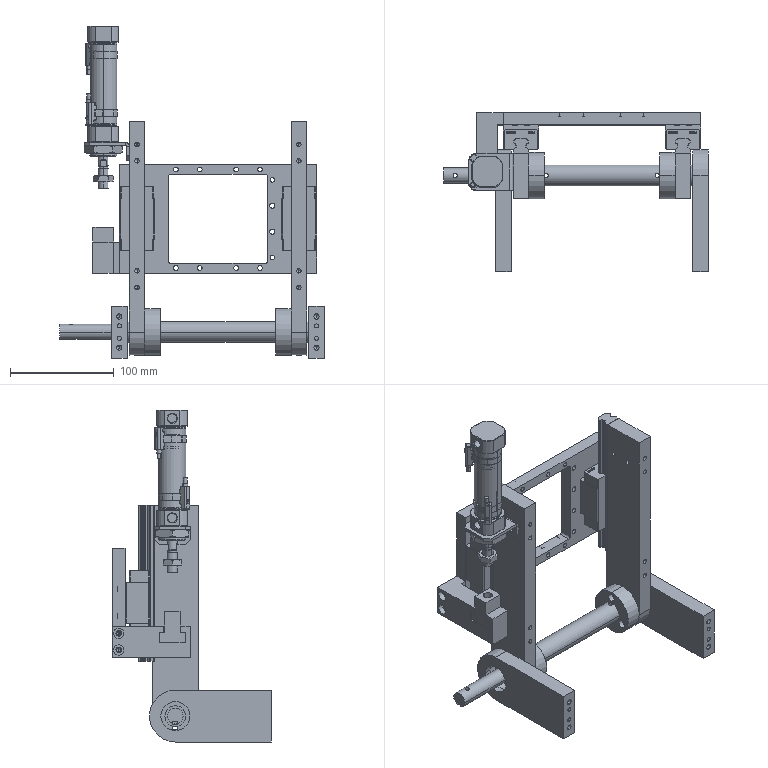Assembly | SolidWorks | mm | 21 component files | 21 solids | 1697 faces | box 255 x 153.1 x 320 mm | volume 900386 mm3 | plane 917 | cylinder 430 | spline 214 | cone 116 | torus 16 | sphere 4 | commonest cylinder face diameters 4.5 x60 4.2 x44 8 x36 4 x34 0.8 x32 3.3 x16 26.4 x16 3.24 x16
Bill of materials:
02 | 2 |  | Thick rectangular bar with one fully rounded end. A large through-bore runs near the rounded end, and the flat square end has small holes.
03 | 1 |  | Stepped cylindrical shaft with a larger central section and smaller-diameter ends, plus small radial cross-holes.
04 | 2 |  | Long flat bar or arm with one rounded end. The rounded end has a bore with a keyway and three small holes around it, and more small holes run along the bar.
05 | 1 |  | Flat rectangular plate with a large rounded-corner rectangular cutout off-center, and many through-holes spread around it.
14 | 1 |  | Bent L-shaped bracket of uniform thickness. One flange has a large circular hole, the other has two smaller holes, and the free corners are chamfered.
15 | 1 |  | Rectangular block with a T-shaped (undercut) stepped slot cut through one end region. Two through-holes sit at the opposite end.
18 | 2 |  | Thick circular disk or hub with a central bore that has a rectangular keyway, and three equally spaced axial holes.
19 | 1 |  | T-profile block: a wider base flange with chamfered edges under a narrower rectangular upright, with a single round hole entering from the top.
CS1_M_S25 | 2 |  | Thin flat strip formed into a near-circular loop. Its ends meet at a small block-shaped body that carries a stepped cylindrical pin on top and a domed boss on one side.
MF_25x50_S_U_c | 1 |  | Cylindrical rod with an eight-sided prismatic head at one end and an eight-sided collar near the other end, which then ends in a short cylindrical stub.
MF_25x50_S_U_r | 1 |  | Slender pin with a disk-shaped head carrying a circumferential groove. Near the far end the shaft has a short reduced or flattened section before a smaller end stub.
MF25_M10x1_25_Nut | 1 |  | Low-profile hexagonal nut shape with a central round bore and chamfered corners on both faces.
MF25_M26x1_5_Nut | 1 |  | Thin hexagonal ring: a flat six-sided body with a large central circular bore and chamfered hex corners on both faces, shaped like a thin hex nut.
SlideRailHIWINHG15R150-C | 2 |  | Long straight prismatic bar with a constant shaped cross-section: rounded concave grooves near the top of each side, a narrow waist, and a wider base with chamfered corners. Three round through holes are spaced along its length.
SliderHIWINHGH15CA-C | 2 |  | Rectangular block with a lengthwise channel open on one face. The channel has rounded lobes on both side walls. The outer shape is stepped, and a small cylindrical stub sticks out from one end.
Mates:
1. distance | 02-1 face at (-79.5, -66.3, 30) dir (1, 0, 0) | 04-1 face at (-77.5, -32.5, 131.5) dir (-1, 0, 0)
2. concentric | 03-1 face at (110.5, -32.5, 30) dir (-1, 0, 0) r 10 | 02-1 face at (-79.5, -32.5, 30) dir (-1, 0, 0) r 14
3. concentric | 03-1 face at (110.5, -32.5, 30) dir (-1, 0, 0) r 10 | 04-1 face at (-77.5, -32.5, 30) dir (1, 0, 0) r 10
4. coincident | 03-1 face at (-49.5, -35, 17) dir (0, 1, 0) | 04-1 face at (-77.5, -35, 24) dir (0, 1, 0)
5. coincident | 15-1 face at (-113, -42, 100.8) dir (0, 0, 1) | 19-1 face at (-102.5, -29.5, 100.8) dir (0, 0, -1)
6. parallel | 15-1 face at (-93, -9.5, 101.8) dir (1, 0, 0) | 19-1 face at (-92.5, -17, 110.8) dir (1, 0, 0)
7. coincident | 04-1 face at (-77.5, -32.5, 131.5) dir (-1, 0, 0) | 14-1 face at (-77.5, -47, 195) dir (1, 0, 0)
8. coincident | 04-1 face at (-70, -12, 131.5) dir (0, 1, 0) | 14-1 face at (-81.237, -12, 213) dir (0, 1, 0)
9. distance | 14-1 face at (-80.5, -47, 213) dir (0, 0, 1) | 04-1 face at (-62.5, -10, 233) dir (0, 0, 1)
10. coincident | 14-1 face at (-80.5, -47, 213) dir (0, 0, 1) | MF_25x50_S_U_M_2_0-1/MF_25x50_S_U_c-1 face at (-102.5, -29.5, 213) dir (0, 0, -1)
11. concentric | 14-1 face at (-102.5, -29.5, 213) dir (0, 0, -1) r 13 | MF_25x50_S_U_M_2_0-1/MF_25x50_S_U_c-1 face at (-102.5, -29.5, 213) dir (0, 0, -1) r 13
12. concentric | 19-1 face at (-102.5, -29.5, 130.8) dir (0, 0, 1) r 4.4 | MF_25x50_S_U_M_2_0-1/MF_25x50_S_U_r-1 face at (-102.5, -29.5, 301) dir (0, 0, -1) r 5
13. coincident | 04-1 face at (-70, -12, 131.5) dir (0, 1, 0) | SlideRailHIWINHG15R150-C-1 face at (-76.8, -12, 83) dir (0, -1, 0)
14. coincident | 04-1 face at (-77.5, -12, 83) dir (0, 0, 1) | SlideRailHIWINHG15R150-C-1 face at (-70, 3, 83) dir (0, 0, -1)
15. coincident | 04-1 face at (-77.5, -32.5, 131.5) dir (-1, 0, 0) | SlideRailHIWINHG15R150-C-1 face at (-77.5, -8.757, 83) dir (-1, 0, 0)
16. coincident | SlideRailHIWINHG15R150-C-1 face at (-64.951, 3, 83) dir (0, 1, 0) | SliderHIWINHGH15CA-C-1 face at (-75.049, 3, 119.6) dir (0, -1, 0)
17. coincident | SlideRailHIWINHG15R150-C-1 plane at (-70, 3, 158) dir (1, 0, 0) | SliderHIWINHGH15CA-C-1 plane at (-70, 3, 139.3) dir (1, 0, 0)
18. distance | SlideRailHIWINHG15R150-C-1 face at (-70, 3, 233) dir (0, 0, 1) | SliderHIWINHGH15CA-C-1 face at (-70, 3, 170) dir (0, 0, 1)
19. coincident | 05-1 face at (-87, 28, 86.8) dir (-1, 0, 0) | 15-1 face at (-87, -9.5, 101.8) dir (1, 0, 0)
20. coincident | 05-1 face at (-87, 28, 86.8) dir (0, 0, -1) | 15-1 face at (-113, 28, 86.8) dir (0, 0, -1)
21. coincident | 05-1 face at (8, 28, 139.3) dir (0, 1, 0) | 15-1 face at (-113, 28, 86.8) dir (0, 1, 0)
22. coincident | 05-1 face at (8, 16, 139.3) dir (0, -1, 0) | SliderHIWINHGH15CA-C-1 face at (-79, 16, 119.6) dir (0, 1, 0)
23. coincident | 05-1 plane at (8, 22, 139.3) dir (0, 0, 1) | SliderHIWINHGH15CA-C-1 plane at (-70, 3, 139.3) dir (0, 0, 1)
24. coincident | 05-1 face at (-87, 28, 86.8) dir (-1, 0, 0) | SliderHIWINHGH15CA-C-1 face at (-87, 15, 119.6) dir (-1, 0, 0)
25. coincident | SliderHIWINHGH15CA-C-1 face at (-70, 3, 170) dir (0, 0, 1) | SliderHIWINHGH15CA-C-2 face at (86, 3, 170) dir (0, 0, 1)
26. coincident | 05-1 face at (103, 28, 86.8) dir (1, 0, 0) | SliderHIWINHGH15CA-C-2 face at (103, 10, 119.6) dir (1, 0, 0)
27. coincident | 04-1 face at (-77.5, -12, 83) dir (0, 0, 1) | SlideRailHIWINHG15R150-C-2 face at (86, 3, 83) dir (0, 0, -1)
28. coincident | SlideRailHIWINHG15R150-C-2 face at (91.049, 3, 83) dir (0, 1, 0) | SliderHIWINHGH15CA-C-2 face at (80.951, 3, 119.6) dir (0, -1, 0)
29. coincident | SlideRailHIWINHG15R150-C-2 plane at (86, 3, 158) dir (1, 0, 0) | SliderHIWINHGH15CA-C-2 plane at (86, 3, 139.3) dir (1, 0, 0)
30. coincident | 04-2 face at (93.5, -10, 233) dir (0, 1, 0) | 04-1 face at (-62.5, -10, 233) dir (0, 1, 0)
31. concentric | 03-1 face at (110.5, -32.5, 30) dir (-1, 0, 0) r 10 | 04-2 face at (78.5, -32.5, 30) dir (1, 0, 0) r 10
32. coincident | 04-2 face at (86, -12, 131.5) dir (0, 1, 0) | SlideRailHIWINHG15R150-C-2 face at (79.2, -12, 83) dir (0, -1, 0)
33. coincident | 04-2 face at (78.5, -32.5, 131.5) dir (-1, 0, 0) | SlideRailHIWINHG15R150-C-2 face at (78.5, -8.757, 83) dir (-1, 0, 0)
34. concentric | 03-1 face at (110.5, -32.5, 30) dir (-1, 0, 0) r 10 | 18-1 face at (78.5, -32.5, 30) dir (-1, 0, 0) r 10
35. coincident | 04-2 face at (78.5, -32.5, 131.5) dir (-1, 0, 0) | 18-1 face at (78.5, -32.5, 30) dir (1, 0, 0)
36. coincident | 04-2 face at (78.5, -30, 24) dir (0, -1, 0) | 18-1 face at (63.5, -30, 22) dir (0, -1, 0)
37. concentric | 02-2 face at (95.5, -32.5, 30) dir (1, 0, 0) r 14 | 03-1 face at (110.5, -32.5, 30) dir (-1, 0, 0) r 10
38. coincident | 03-1 face at (110.5, -32.5, 30) dir (1, 0, 0) | 02-2 face at (110.5, -66.3, 30) dir (1, 0, 0)
39. distance | 02-2 face at (95.5, -66.3, 30) dir (-1, 0, 0) | 04-2 face at (93.5, -32.5, 131.5) dir (1, 0, 0)
40. coincident | 04-1 face at (-62.5, -32.5, 131.5) dir (1, 0, 0) | 18-2 face at (-62.5, -32.5, 30) dir (-1, 0, 0)
41. coincident | 04-1 face at (-77.5, -30, 24) dir (0, -1, 0) | 18-2 face at (-47.5, -30, 22) dir (0, -1, 0)
42. concentric | 03-1 face at (110.5, -32.5, 30) dir (-1, 0, 0) r 10 | 18-2 face at (-62.5, -32.5, 30) dir (1, 0, 0) r 10
43. coincident | MF_25x50_S_U_c-1 axis at (-80.9, 0, 0) dir (1, 0, 0) | MF_25x50_S_U_r-1 axis at (-80.9, 0, 0) dir (1, 0, 0)
44. coincident | MF_25x50_S_U_c-1 axis at (-80.9, 0, 0) dir (1, 0, 0) | MF_25x50_S_U_r-1 axis at (-80.9, 0, 0) dir (1, 0, 0)
45. coincident | MF_25x50_S_U_c-1 axis at (-80.9, 0, 0) dir (1, 0, 0) | MF_25x50_S_U_r-1 axis at (-80.9, 0, 0) dir (1, 0, 0)
46. angle | MF_25x50_S_U_r-1 plane at (0, 0, 0) dir (0, 0, -1) | MF_25x50_S_U_c-1 plane at (0, 0, 0) dir (0, 0, -1)